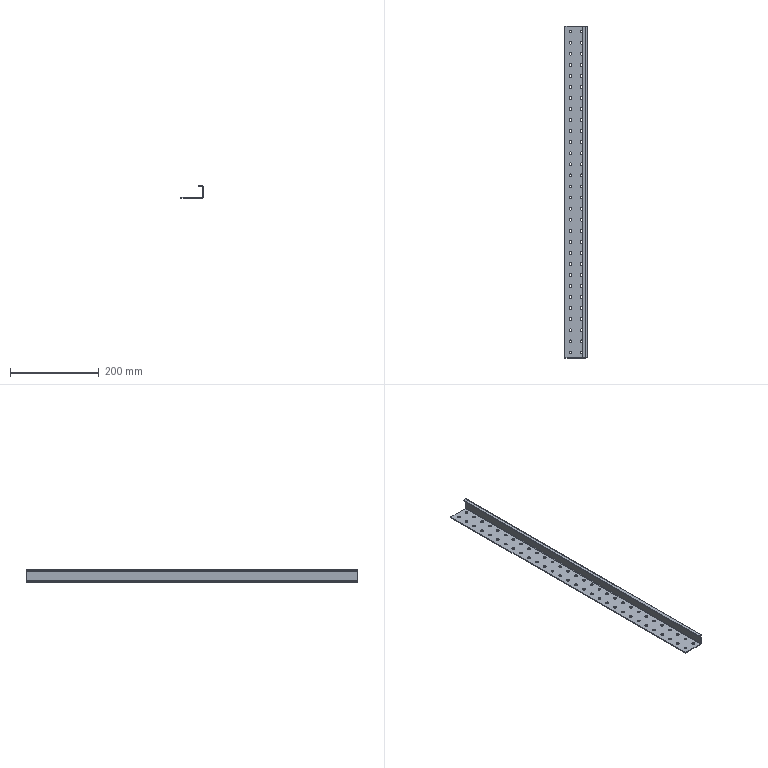Component | SolidWorks | Baffle(No.24)-1 | 1 solid | 142 faces | volume 120193 mm3 | cylinder 124 | plane 18 | commonest cylinder face diameters 6.5 x120 6 x2 2 x2